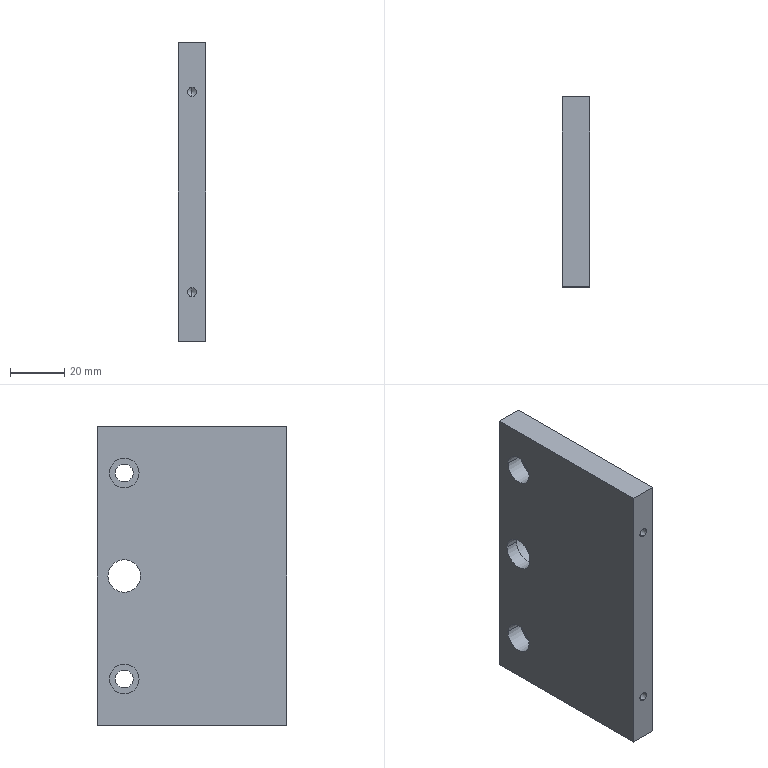Component | SolidWorks | CS021-A10-A003-1 | 1 solid | 29 faces | box 10 x 70 x 110 mm | volume 73715 mm3 | cylinder 16 | plane 9 | cone 4 | commonest cylinder face diameters 11 x4 6.6 x4 3.3 x4 12 x2 16 x2 | material AL6061
build123d program:
from build123d import *

# Parameters (mm, degrees)
SKETCH1_W                                          = 110
SKETCH1_H                                          = 70
BOSS_EXTRUDE1_DEPTH                                = 5
M4_TAPPED_HOLE1_D                                  = 3.3
M4_TAPPED_HOLE1_DEPTH                              = 11.5
M4_TAPPED_HOLE1_TIP                                = 0.9914
HOLE_SIZE_ACCORDING_TO_SLOTTED_PAN_HEA_D           = 6.6
HOLE_SIZE_ACCORDING_TO_SLOTTED_PAN_HEA_CBORE_D     = 11
HOLE_SIZE_ACCORDING_TO_SLOTTED_PAN_HEA_CBORE_DEPTH = 6.8
SKETCH6_R                                          = 8
CUT_EXTRUDE1_DEPTH                                 = 5
SKETCH7_R                                          = 6
CUT_EXTRUDE2_DEPTH                                 = 66.383


with BuildPart() as part:
    # Sketch1 → Boss-Extrude1 (new, symmetric)
    with BuildSketch(Plane(origin=(0, 0, 0), x_dir=(1, 0, 0), z_dir=(0, 1, 0))):
        Rectangle(SKETCH1_W, SKETCH1_H)
    extrude(amount=BOSS_EXTRUDE1_DEPTH, both=True)

    # M4 Tapped Hole1
    with Locations(Plane.XY.offset(35)):
        with Locations((-37, 0), (37, 0)):
            Hole(M4_TAPPED_HOLE1_D / 2, depth=M4_TAPPED_HOLE1_DEPTH)
            with Locations((0, 0, -(M4_TAPPED_HOLE1_DEPTH + M4_TAPPED_HOLE1_TIP / 2))):  # 118° drill point
                Cone(0, M4_TAPPED_HOLE1_D / 2, M4_TAPPED_HOLE1_TIP, mode=Mode.SUBTRACT)

    # Hole Size _according to_ Slotted Pan Hea (through all)
    with Locations(Plane(origin=(0, 5, 0), x_dir=(1, 0, 0), z_dir=(0, 1, 0))):
        with Locations((-38, 25), (38, 25)):
            CounterBoreHole(HOLE_SIZE_ACCORDING_TO_SLOTTED_PAN_HEA_D / 2, HOLE_SIZE_ACCORDING_TO_SLOTTED_PAN_HEA_CBORE_D / 2, HOLE_SIZE_ACCORDING_TO_SLOTTED_PAN_HEA_CBORE_DEPTH)

    # Sketch6 → Cut-Extrude1 (cut)
    with BuildSketch(Plane.XZ.offset(5)):
        with Locations(Location((0, -25, 0), (0, 0, 270))):
            Circle(SKETCH6_R)
    extrude(amount=-CUT_EXTRUDE1_DEPTH, mode=Mode.SUBTRACT)

    # Sketch7 → Cut-Extrude2 (cut, through all)
    with BuildSketch(Plane.XZ):
        with Locations(Location((0, -25, 0), (0, 0, 270))):
            Circle(SKETCH7_R)
    extrude(amount=-CUT_EXTRUDE2_DEPTH, mode=Mode.SUBTRACT)


solid = part.part

# Placed as in the assembly
solid = solid.moved(Location((-159.051, 59.817, 0), (90, 0, 90)))
STEP:
#1=COLOUR_RGB('',0.7922,0.8196,0.9333);
#2=FILL_AREA_STYLE_COLOUR('',#1);
#3=FILL_AREA_STYLE('',(#2));
#4=SURFACE_STYLE_FILL_AREA(#3);
#5=SURFACE_SIDE_STYLE('',(#4));
#6=SURFACE_STYLE_USAGE(.BOTH.,#5);
#7=PRESENTATION_STYLE_ASSIGNMENT((#6));
#8=CARTESIAN_POINT('',(-6.459,3.103,-0.));
#9=VERTEX_POINT('',#8);
#10=CARTESIAN_POINT('',(-6.459,3.575,-0.));
#11=VERTEX_POINT('',#10);
#12=CARTESIAN_POINT('',(-6.459,3.339,-0.));
#13=DIRECTION('',(1.,-0.,0.));
#14=DIRECTION('',(0.,1.,0.));
#15=AXIS2_PLACEMENT_3D('',#12,#13,#14);
#16=CIRCLE('',#15,0.2362);
#17=EDGE_CURVE('',#9,#11,#16,.T.);
#18=ORIENTED_EDGE('',*,*,#17,.F.);
#19=CARTESIAN_POINT('',(-6.262,3.103,-0.));
#20=VERTEX_POINT('',#19);
#21=CARTESIAN_POINT('',(-6.459,3.103,-0.));
#22=DIRECTION('',(1.,-0.,0.));
#23=VECTOR('',#22,39.37);
#24=LINE('',#21,#23);
#25=EDGE_CURVE('',#9,#20,#24,.T.);
#26=ORIENTED_EDGE('',*,*,#25,.T.);
#27=CARTESIAN_POINT('',(-6.262,3.575,-0.));
#28=VERTEX_POINT('',#27);
#29=CARTESIAN_POINT('',(-6.262,3.339,-0.));
#30=DIRECTION('',(1.,-0.,0.));
#31=DIRECTION('',(0.,1.,0.));
#32=AXIS2_PLACEMENT_3D('',#29,#30,#31);
#33=CIRCLE('',#32,0.2362);
#34=EDGE_CURVE('',#20,#28,#33,.T.);
#35=ORIENTED_EDGE('',*,*,#34,.T.);
#36=CARTESIAN_POINT('',(-6.459,3.575,-0.));
#37=DIRECTION('',(1.,-0.,0.));
#38=VECTOR('',#37,39.37);
#39=LINE('',#36,#38);
#40=EDGE_CURVE('',#11,#28,#39,.T.);
#41=ORIENTED_EDGE('',*,*,#40,.F.);
#42=EDGE_LOOP('',(#18,#26,#35,#41));
#43=FACE_OUTER_BOUND('',#42,.T.);
#44=CARTESIAN_POINT('',(-6.459,3.339,-0.));
#45=DIRECTION('',(1.,-0.,0.));
#46=DIRECTION('',(0.,1.,0.));
#47=AXIS2_PLACEMENT_3D('',#44,#45,#46);
#48=CYLINDRICAL_SURFACE('',#47,0.2362);
#49=ADVANCED_FACE('',(#43),#48,.F.);
#50=CARTESIAN_POINT('',(-6.262,3.024,-0.));
#51=VERTEX_POINT('',#50);
#52=CARTESIAN_POINT('',(-6.262,3.654,-0.));
#53=VERTEX_POINT('',#52);
#54=CARTESIAN_POINT('',(-6.262,3.339,-0.));
#55=DIRECTION('',(1.,-0.,0.));
#56=DIRECTION('',(0.,1.,0.));
#57=AXIS2_PLACEMENT_3D('',#54,#55,#56);
#58=CIRCLE('',#57,0.315);
#59=EDGE_CURVE('',#51,#53,#58,.T.);
#60=ORIENTED_EDGE('',*,*,#59,.F.);
#61=CARTESIAN_POINT('',(-6.065,3.024,-0.));
#62=VERTEX_POINT('',#61);
#63=CARTESIAN_POINT('',(-6.262,3.024,-0.));
#64=DIRECTION('',(1.,-0.,0.));
#65=VECTOR('',#64,39.37);
#66=LINE('',#63,#65);
#67=EDGE_CURVE('',#51,#62,#66,.T.);
#68=ORIENTED_EDGE('',*,*,#67,.T.);
#69=CARTESIAN_POINT('',(-6.065,3.654,-0.));
#70=VERTEX_POINT('',#69);
#71=CARTESIAN_POINT('',(-6.065,3.339,-0.));
#72=DIRECTION('',(1.,-0.,0.));
#73=DIRECTION('',(0.,1.,0.));
#74=AXIS2_PLACEMENT_3D('',#71,#72,#73);
#75=CIRCLE('',#74,0.315);
#76=EDGE_CURVE('',#62,#70,#75,.T.);
#77=ORIENTED_EDGE('',*,*,#76,.T.);
#78=CARTESIAN_POINT('',(-6.262,3.654,-0.));
#79=DIRECTION('',(1.,-0.,0.));
#80=VECTOR('',#79,39.37);
#81=LINE('',#78,#80);
#82=EDGE_CURVE('',#53,#70,#81,.T.);
#83=ORIENTED_EDGE('',*,*,#82,.F.);
#84=EDGE_LOOP('',(#60,#68,#77,#83));
#85=FACE_OUTER_BOUND('',#84,.T.);
#86=CARTESIAN_POINT('',(-6.262,3.339,-0.));
#87=DIRECTION('',(1.,-0.,0.));
#88=DIRECTION('',(0.,1.,0.));
#89=AXIS2_PLACEMENT_3D('',#86,#87,#88);
#90=CYLINDRICAL_SURFACE('',#89,0.315);
#91=ADVANCED_FACE('',(#85),#90,.F.);
#92=CARTESIAN_POINT('',(-6.191,3.556,-1.496));
#93=VERTEX_POINT('',#92);
#94=CARTESIAN_POINT('',(-6.191,3.123,-1.496));
#95=VERTEX_POINT('',#94);
#96=CARTESIAN_POINT('',(-6.191,3.339,-1.496));
#97=DIRECTION('',(-1.,0.,0.));
#98=DIRECTION('',(0.,-1.,0.));
#99=AXIS2_PLACEMENT_3D('',#96,#97,#98);
#100=CIRCLE('',#99,0.2165);
#101=EDGE_CURVE('',#93,#95,#100,.T.);
#102=ORIENTED_EDGE('',*,*,#101,.F.);
#103=CARTESIAN_POINT('',(-6.459,3.556,-1.496));
#104=VERTEX_POINT('',#103);
#105=CARTESIAN_POINT('',(-6.459,3.556,-1.496));
#106=DIRECTION('',(-1.,0.,0.));
#107=VECTOR('',#106,39.37);
#108=LINE('',#105,#107);
#109=EDGE_CURVE('',#93,#104,#108,.T.);
#110=ORIENTED_EDGE('',*,*,#109,.T.);
#111=CARTESIAN_POINT('',(-6.459,3.123,-1.496));
#112=VERTEX_POINT('',#111);
#113=CARTESIAN_POINT('',(-6.459,3.339,-1.496));
#114=DIRECTION('',(-1.,0.,0.));
#115=DIRECTION('',(0.,-1.,0.));
#116=AXIS2_PLACEMENT_3D('',#113,#114,#115);
#117=CIRCLE('',#116,0.2165);
#118=EDGE_CURVE('',#104,#112,#117,.T.);
#119=ORIENTED_EDGE('',*,*,#118,.T.);
#120=CARTESIAN_POINT('',(-6.459,3.123,-1.496));
#121=DIRECTION('',(-1.,0.,0.));
#122=VECTOR('',#121,39.37);
#123=LINE('',#120,#122);
#124=EDGE_CURVE('',#95,#112,#123,.T.);
#125=ORIENTED_EDGE('',*,*,#124,.F.);
#126=EDGE_LOOP('',(#102,#110,#119,#125));
#127=FACE_OUTER_BOUND('',#126,.T.);
#128=CARTESIAN_POINT('',(-6.459,3.339,-1.496));
#129=DIRECTION('',(-1.,0.,0.));
#130=DIRECTION('',(0.,-1.,0.));
#131=AXIS2_PLACEMENT_3D('',#128,#129,#130);
#132=CYLINDRICAL_SURFACE('',#131,0.2165);
#133=ADVANCED_FACE('',(#127),#132,.F.);
#134=CARTESIAN_POINT('',(-6.065,3.469,-1.496));
#135=VERTEX_POINT('',#134);
#136=CARTESIAN_POINT('',(-6.065,3.209,-1.496));
#137=VERTEX_POINT('',#136);
#138=CARTESIAN_POINT('',(-6.065,3.339,-1.496));
#139=DIRECTION('',(-1.,0.,0.));
#140=DIRECTION('',(0.,-1.,0.));
#141=AXIS2_PLACEMENT_3D('',#138,#139,#140);
#142=CIRCLE('',#141,0.1299);
#143=EDGE_CURVE('',#135,#137,#142,.T.);
#144=ORIENTED_EDGE('',*,*,#143,.F.);
#145=CARTESIAN_POINT('',(-6.191,3.469,-1.496));
#146=VERTEX_POINT('',#145);
#147=CARTESIAN_POINT('',(-6.459,3.469,-1.496));
#148=DIRECTION('',(-1.,0.,0.));
#149=VECTOR('',#148,39.37);
#150=LINE('',#147,#149);
#151=EDGE_CURVE('',#135,#146,#150,.T.);
#152=ORIENTED_EDGE('',*,*,#151,.T.);
#153=CARTESIAN_POINT('',(-6.191,3.209,-1.496));
#154=VERTEX_POINT('',#153);
#155=CARTESIAN_POINT('',(-6.191,3.339,-1.496));
#156=DIRECTION('',(-1.,0.,0.));
#157=DIRECTION('',(0.,-1.,0.));
#158=AXIS2_PLACEMENT_3D('',#155,#156,#157);
#159=CIRCLE('',#158,0.1299);
#160=EDGE_CURVE('',#146,#154,#159,.T.);
#161=ORIENTED_EDGE('',*,*,#160,.T.);
#162=CARTESIAN_POINT('',(-6.459,3.209,-1.496));
#163=DIRECTION('',(-1.,0.,0.));
#164=VECTOR('',#163,39.37);
#165=LINE('',#162,#164);
#166=EDGE_CURVE('',#137,#154,#165,.T.);
#167=ORIENTED_EDGE('',*,*,#166,.F.);
#168=EDGE_LOOP('',(#144,#152,#161,#167));
#169=FACE_OUTER_BOUND('',#168,.T.);
#170=CARTESIAN_POINT('',(-6.459,3.339,-1.496));
#171=DIRECTION('',(-1.,0.,0.));
#172=DIRECTION('',(0.,-1.,0.));
#173=AXIS2_PLACEMENT_3D('',#170,#171,#172);
#174=CYLINDRICAL_SURFACE('',#173,0.1299);
#175=ADVANCED_FACE('',(#169),#174,.F.);
#176=CARTESIAN_POINT('',(-6.191,3.556,1.496));
#177=VERTEX_POINT('',#176);
#178=CARTESIAN_POINT('',(-6.191,3.123,1.496));
#179=VERTEX_POINT('',#178);
#180=CARTESIAN_POINT('',(-6.191,3.339,1.496));
#181=DIRECTION('',(-1.,0.,0.));
#182=DIRECTION('',(0.,-1.,0.));
#183=AXIS2_PLACEMENT_3D('',#180,#181,#182);
#184=CIRCLE('',#183,0.2165);
#185=EDGE_CURVE('',#177,#179,#184,.T.);
#186=ORIENTED_EDGE('',*,*,#185,.F.);
#187=CARTESIAN_POINT('',(-6.459,3.556,1.496));
#188=VERTEX_POINT('',#187);
#189=CARTESIAN_POINT('',(-6.459,3.556,1.496));
#190=DIRECTION('',(-1.,0.,0.));
#191=VECTOR('',#190,39.37);
#192=LINE('',#189,#191);
#193=EDGE_CURVE('',#177,#188,#192,.T.);
#194=ORIENTED_EDGE('',*,*,#193,.T.);
#195=CARTESIAN_POINT('',(-6.459,3.123,1.496));
#196=VERTEX_POINT('',#195);
#197=CARTESIAN_POINT('',(-6.459,3.339,1.496));
#198=DIRECTION('',(-1.,0.,0.));
#199=DIRECTION('',(0.,-1.,0.));
#200=AXIS2_PLACEMENT_3D('',#197,#198,#199);
#201=CIRCLE('',#200,0.2165);
#202=EDGE_CURVE('',#188,#196,#201,.T.);
#203=ORIENTED_EDGE('',*,*,#202,.T.);
#204=CARTESIAN_POINT('',(-6.459,3.123,1.496));
#205=DIRECTION('',(-1.,0.,0.));
#206=VECTOR('',#205,39.37);
#207=LINE('',#204,#206);
#208=EDGE_CURVE('',#179,#196,#207,.T.);
#209=ORIENTED_EDGE('',*,*,#208,.F.);
#210=EDGE_LOOP('',(#186,#194,#203,#209));
#211=FACE_OUTER_BOUND('',#210,.T.);
#212=CARTESIAN_POINT('',(-6.459,3.339,1.496));
#213=DIRECTION('',(-1.,0.,0.));
#214=DIRECTION('',(0.,-1.,0.));
#215=AXIS2_PLACEMENT_3D('',#212,#213,#214);
#216=CYLINDRICAL_SURFACE('',#215,0.2165);
#217=ADVANCED_FACE('',(#211),#216,.F.);
#218=CARTESIAN_POINT('',(-6.065,3.469,1.496));
#219=VERTEX_POINT('',#218);
#220=CARTESIAN_POINT('',(-6.065,3.209,1.496));
#221=VERTEX_POINT('',#220);
#222=CARTESIAN_POINT('',(-6.065,3.339,1.496));
#223=DIRECTION('',(-1.,0.,0.));
#224=DIRECTION('',(0.,-1.,0.));
#225=AXIS2_PLACEMENT_3D('',#222,#223,#224);
#226=CIRCLE('',#225,0.1299);
#227=EDGE_CURVE('',#219,#221,#226,.T.);
#228=ORIENTED_EDGE('',*,*,#227,.F.);
#229=CARTESIAN_POINT('',(-6.191,3.469,1.496));
#230=VERTEX_POINT('',#229);
#231=CARTESIAN_POINT('',(-6.459,3.469,1.496));
#232=DIRECTION('',(-1.,0.,0.));
#233=VECTOR('',#232,39.37);
#234=LINE('',#231,#233);
#235=EDGE_CURVE('',#219,#230,#234,.T.);
#236=ORIENTED_EDGE('',*,*,#235,.T.);
#237=CARTESIAN_POINT('',(-6.191,3.209,1.496));
#238=VERTEX_POINT('',#237);
#239=CARTESIAN_POINT('',(-6.191,3.339,1.496));
#240=DIRECTION('',(-1.,0.,0.));
#241=DIRECTION('',(0.,-1.,0.));
#242=AXIS2_PLACEMENT_3D('',#239,#240,#241);
#243=CIRCLE('',#242,0.1299);
#244=EDGE_CURVE('',#230,#238,#243,.T.);
#245=ORIENTED_EDGE('',*,*,#244,.T.);
#246=CARTESIAN_POINT('',(-6.459,3.209,1.496));
#247=DIRECTION('',(-1.,0.,0.));
#248=VECTOR('',#247,39.37);
#249=LINE('',#246,#248);
#250=EDGE_CURVE('',#221,#238,#249,.T.);
#251=ORIENTED_EDGE('',*,*,#250,.F.);
#252=EDGE_LOOP('',(#228,#236,#245,#251));
#253=FACE_OUTER_BOUND('',#252,.T.);
#254=CARTESIAN_POINT('',(-6.459,3.339,1.496));
#255=DIRECTION('',(-1.,0.,0.));
#256=DIRECTION('',(0.,-1.,0.));
#257=AXIS2_PLACEMENT_3D('',#254,#255,#256);
#258=CYLINDRICAL_SURFACE('',#257,0.1299);
#259=ADVANCED_FACE('',(#253),#258,.F.);
#260=CARTESIAN_POINT('',(-6.262,1.43,-1.522));
#261=VERTEX_POINT('',#260);
#262=CARTESIAN_POINT('',(-6.262,1.43,-1.392));
#263=VERTEX_POINT('',#262);
#264=CARTESIAN_POINT('',(-6.262,1.43,-1.457));
#265=DIRECTION('',(-0.,-1.,-0.));
#266=DIRECTION('',(0.,0.,1.));
#267=AXIS2_PLACEMENT_3D('',#264,#265,#266);
#268=CIRCLE('',#267,0.06496);
#269=EDGE_CURVE('',#261,#263,#268,.T.);
#270=ORIENTED_EDGE('',*,*,#269,.F.);
#271=CARTESIAN_POINT('',(-6.262,0.977,-1.522));
#272=VERTEX_POINT('',#271);
#273=CARTESIAN_POINT('',(-6.262,0.977,-1.522));
#274=DIRECTION('',(-0.,-1.,-0.));
#275=VECTOR('',#274,39.37);
#276=LINE('',#273,#275);
#277=EDGE_CURVE('',#261,#272,#276,.T.);
#278=ORIENTED_EDGE('',*,*,#277,.T.);
#279=CARTESIAN_POINT('',(-6.262,0.977,-1.392));
#280=VERTEX_POINT('',#279);
#281=CARTESIAN_POINT('',(-6.262,0.977,-1.457));
#282=DIRECTION('',(-0.,-1.,-0.));
#283=DIRECTION('',(0.,0.,1.));
#284=AXIS2_PLACEMENT_3D('',#281,#282,#283);
#285=CIRCLE('',#284,0.06496);
#286=EDGE_CURVE('',#272,#280,#285,.T.);
#287=ORIENTED_EDGE('',*,*,#286,.T.);
#288=CARTESIAN_POINT('',(-6.262,0.977,-1.392));
#289=DIRECTION('',(-0.,-1.,-0.));
#290=VECTOR('',#289,39.37);
#291=LINE('',#288,#290);
#292=EDGE_CURVE('',#263,#280,#291,.T.);
#293=ORIENTED_EDGE('',*,*,#292,.F.);
#294=EDGE_LOOP('',(#270,#278,#287,#293));
#295=FACE_OUTER_BOUND('',#294,.T.);
#296=CARTESIAN_POINT('',(-6.262,0.977,-1.457));
#297=DIRECTION('',(-0.,-1.,-0.));
#298=DIRECTION('',(0.,0.,1.));
#299=AXIS2_PLACEMENT_3D('',#296,#297,#298);
#300=CYLINDRICAL_SURFACE('',#299,0.06496);
#301=ADVANCED_FACE('',(#295),#300,.F.);
#302=CARTESIAN_POINT('',(-6.262,1.469,-1.457));
#303=VERTEX_POINT('',#302);
#304=CARTESIAN_POINT('',(-6.262,1.43,-1.392));
#305=DIRECTION('',(-0.,-0.515,0.8572));
#306=VECTOR('',#305,39.37);
#307=LINE('',#304,#306);
#308=EDGE_CURVE('',#303,#263,#307,.T.);
#309=ORIENTED_EDGE('',*,*,#308,.F.);
#310=CARTESIAN_POINT('',(-6.262,1.43,-1.522));
#311=DIRECTION('',(-0.,-0.515,-0.8572));
#312=VECTOR('',#311,39.37);
#313=LINE('',#310,#312);
#314=EDGE_CURVE('',#303,#261,#313,.T.);
#315=ORIENTED_EDGE('',*,*,#314,.T.);
#316=ORIENTED_EDGE('',*,*,#269,.T.);
#317=EDGE_LOOP('',(#309,#315,#316));
#318=FACE_OUTER_BOUND('',#317,.T.);
#319=CARTESIAN_POINT('',(-6.262,1.43,-1.457));
#320=DIRECTION('',(-0.,-1.,-0.));
#321=DIRECTION('',(0.,0.,1.));
#322=AXIS2_PLACEMENT_3D('',#319,#320,#321);
#323=CONICAL_SURFACE('',#322,0.06496,1.03);
#324=ADVANCED_FACE('',(#318),#323,.F.);
#325=CARTESIAN_POINT('',(-6.262,1.43,1.392));
#326=VERTEX_POINT('',#325);
#327=CARTESIAN_POINT('',(-6.262,1.43,1.522));
#328=VERTEX_POINT('',#327);
#329=CARTESIAN_POINT('',(-6.262,1.43,1.457));
#330=DIRECTION('',(-0.,-1.,-0.));
#331=DIRECTION('',(0.,0.,1.));
#332=AXIS2_PLACEMENT_3D('',#329,#330,#331);
#333=CIRCLE('',#332,0.06496);
#334=EDGE_CURVE('',#326,#328,#333,.T.);
#335=ORIENTED_EDGE('',*,*,#334,.F.);
#336=CARTESIAN_POINT('',(-6.262,0.977,1.392));
#337=VERTEX_POINT('',#336);
#338=CARTESIAN_POINT('',(-6.262,0.977,1.392));
#339=DIRECTION('',(-0.,-1.,-0.));
#340=VECTOR('',#339,39.37);
#341=LINE('',#338,#340);
#342=EDGE_CURVE('',#326,#337,#341,.T.);
#343=ORIENTED_EDGE('',*,*,#342,.T.);
#344=CARTESIAN_POINT('',(-6.262,0.977,1.522));
#345=VERTEX_POINT('',#344);
#346=CARTESIAN_POINT('',(-6.262,0.977,1.457));
#347=DIRECTION('',(-0.,-1.,-0.));
#348=DIRECTION('',(0.,0.,1.));
#349=AXIS2_PLACEMENT_3D('',#346,#347,#348);
#350=CIRCLE('',#349,0.06496);
#351=EDGE_CURVE('',#337,#345,#350,.T.);
#352=ORIENTED_EDGE('',*,*,#351,.T.);
#353=CARTESIAN_POINT('',(-6.262,0.977,1.522));
#354=DIRECTION('',(-0.,-1.,-0.));
#355=VECTOR('',#354,39.37);
#356=LINE('',#353,#355);
#357=EDGE_CURVE('',#328,#345,#356,.T.);
#358=ORIENTED_EDGE('',*,*,#357,.F.);
#359=EDGE_LOOP('',(#335,#343,#352,#358));
#360=FACE_OUTER_BOUND('',#359,.T.);
#361=CARTESIAN_POINT('',(-6.262,0.977,1.457));
#362=DIRECTION('',(-0.,-1.,-0.));
#363=DIRECTION('',(0.,0.,1.));
#364=AXIS2_PLACEMENT_3D('',#361,#362,#363);
#365=CYLINDRICAL_SURFACE('',#364,0.06496);
#366=ADVANCED_FACE('',(#360),#365,.F.);
#367=CARTESIAN_POINT('',(-6.262,1.469,1.457));
#368=VERTEX_POINT('',#367);
#369=CARTESIAN_POINT('',(-6.262,1.43,1.522));
#370=DIRECTION('',(-0.,-0.515,0.8572));
#371=VECTOR('',#370,39.37);
#372=LINE('',#369,#371);
#373=EDGE_CURVE('',#368,#328,#372,.T.);
#374=ORIENTED_EDGE('',*,*,#373,.F.);
#375=CARTESIAN_POINT('',(-6.262,1.43,1.392));
#376=DIRECTION('',(-0.,-0.515,-0.8572));
#377=VECTOR('',#376,39.37);
#378=LINE('',#375,#377);
#379=EDGE_CURVE('',#368,#326,#378,.T.);
#380=ORIENTED_EDGE('',*,*,#379,.T.);
#381=ORIENTED_EDGE('',*,*,#334,.T.);
#382=EDGE_LOOP('',(#374,#380,#381));
#383=FACE_OUTER_BOUND('',#382,.T.);
#384=CARTESIAN_POINT('',(-6.262,1.43,1.457));
#385=DIRECTION('',(-0.,-1.,-0.));
#386=DIRECTION('',(0.,0.,1.));
#387=AXIS2_PLACEMENT_3D('',#384,#385,#386);
#388=CONICAL_SURFACE('',#387,0.06496,1.03);
#389=ADVANCED_FACE('',(#383),#388,.F.);
#390=CARTESIAN_POINT('',(-6.065,0.977,2.165));
#391=VERTEX_POINT('',#390);
#392=CARTESIAN_POINT('',(-6.065,3.733,2.165));
#393=VERTEX_POINT('',#392);
#394=CARTESIAN_POINT('',(-6.065,0.977,2.165));
#395=DIRECTION('',(0.,1.,0.));
#396=VECTOR('',#395,39.37);
#397=LINE('',#394,#396);
#398=EDGE_CURVE('',#391,#393,#397,.T.);
#399=ORIENTED_EDGE('',*,*,#398,.T.);
#400=CARTESIAN_POINT('',(-6.459,3.733,2.165));
#401=VERTEX_POINT('',#400);
#402=CARTESIAN_POINT('',(-6.459,3.733,2.165));
#403=DIRECTION('',(1.,-0.,0.));
#404=VECTOR('',#403,39.37);
#405=LINE('',#402,#404);
#406=EDGE_CURVE('',#401,#393,#405,.T.);
#407=ORIENTED_EDGE('',*,*,#406,.F.);
#408=CARTESIAN_POINT('',(-6.459,0.977,2.165));
#409=VERTEX_POINT('',#408);
#410=CARTESIAN_POINT('',(-6.459,0.977,2.165));
#411=DIRECTION('',(0.,1.,0.));
#412=VECTOR('',#411,39.37);
#413=LINE('',#410,#412);
#414=EDGE_CURVE('',#409,#401,#413,.T.);
#415=ORIENTED_EDGE('',*,*,#414,.F.);
#416=CARTESIAN_POINT('',(-6.459,0.977,2.165));
#417=DIRECTION('',(1.,-0.,0.));
#418=VECTOR('',#417,39.37);
#419=LINE('',#416,#418);
#420=EDGE_CURVE('',#409,#391,#419,.T.);
#421=ORIENTED_EDGE('',*,*,#420,.T.);
#422=EDGE_LOOP('',(#399,#407,#415,#421));
#423=FACE_OUTER_BOUND('',#422,.T.);
#424=CARTESIAN_POINT('',(-6.459,0.977,2.165));
#425=DIRECTION('',(0.,0.,-1.));
#426=DIRECTION('',(-0.,-1.,-0.));
#427=AXIS2_PLACEMENT_3D('',#424,#425,#426);
#428=PLANE('',#427);
#429=ADVANCED_FACE('',(#423),#428,.F.);
#430=CARTESIAN_POINT('',(-6.065,3.733,-2.165));
#431=VERTEX_POINT('',#430);
#432=CARTESIAN_POINT('',(-6.065,3.733,-2.165));
#433=DIRECTION('',(0.,0.,-1.));
#434=VECTOR('',#433,39.37);
#435=LINE('',#432,#434);
#436=EDGE_CURVE('',#393,#431,#435,.T.);
#437=ORIENTED_EDGE('',*,*,#436,.T.);
#438=CARTESIAN_POINT('',(-6.459,3.733,-2.165));
#439=VERTEX_POINT('',#438);
#440=CARTESIAN_POINT('',(-6.459,3.733,-2.165));
#441=DIRECTION('',(1.,-0.,0.));
#442=VECTOR('',#441,39.37);
#443=LINE('',#440,#442);
#444=EDGE_CURVE('',#439,#431,#443,.T.);
#445=ORIENTED_EDGE('',*,*,#444,.F.);
#446=CARTESIAN_POINT('',(-6.459,3.733,-2.165));
#447=DIRECTION('',(0.,0.,-1.));
#448=VECTOR('',#447,39.37);
#449=LINE('',#446,#448);
#450=EDGE_CURVE('',#401,#439,#449,.T.);
#451=ORIENTED_EDGE('',*,*,#450,.F.);
#452=ORIENTED_EDGE('',*,*,#406,.T.);
#453=EDGE_LOOP('',(#437,#445,#451,#452));
#454=FACE_OUTER_BOUND('',#453,.T.);
#455=CARTESIAN_POINT('',(-6.459,3.733,-2.165));
#456=DIRECTION('',(-0.,-1.,-0.));
#457=DIRECTION('',(-0.,-0.,1.));
#458=AXIS2_PLACEMENT_3D('',#455,#456,#457);
#459=PLANE('',#458);
#460=ADVANCED_FACE('',(#454),#459,.F.);
#461=CARTESIAN_POINT('',(-6.065,0.977,-2.165));
#462=VERTEX_POINT('',#461);
#463=CARTESIAN_POINT('',(-6.065,0.977,-2.165));
#464=DIRECTION('',(-0.,-1.,-0.));
#465=VECTOR('',#464,39.37);
#466=LINE('',#463,#465);
#467=EDGE_CURVE('',#431,#462,#466,.T.);
#468=ORIENTED_EDGE('',*,*,#467,.T.);
#469=CARTESIAN_POINT('',(-6.459,0.977,-2.165));
#470=VERTEX_POINT('',#469);
#471=CARTESIAN_POINT('',(-6.459,0.977,-2.165));
#472=DIRECTION('',(1.,-0.,0.));
#473=VECTOR('',#472,39.37);
#474=LINE('',#471,#473);
#475=EDGE_CURVE('',#470,#462,#474,.T.);
#476=ORIENTED_EDGE('',*,*,#475,.F.);
#477=CARTESIAN_POINT('',(-6.459,0.977,-2.165));
#478=DIRECTION('',(-0.,-1.,-0.));
#479=VECTOR('',#478,39.37);
#480=LINE('',#477,#479);
#481=EDGE_CURVE('',#439,#470,#480,.T.);
#482=ORIENTED_EDGE('',*,*,#481,.F.);
#483=ORIENTED_EDGE('',*,*,#444,.T.);
#484=EDGE_LOOP('',(#468,#476,#482,#483));
#485=FACE_OUTER_BOUND('',#484,.T.);
#486=CARTESIAN_POINT('',(-6.459,0.977,-2.165));
#487=DIRECTION('',(-0.,-0.,1.));
#488=DIRECTION('',(0.,1.,0.));
#489=AXIS2_PLACEMENT_3D('',#486,#487,#488);
#490=PLANE('',#489);
#491=ADVANCED_FACE('',(#485),#490,.F.);
#492=CARTESIAN_POINT('',(-6.262,0.977,-1.457));
#493=DIRECTION('',(-0.,-1.,-0.));
#494=DIRECTION('',(0.,0.,1.));
#495=AXIS2_PLACEMENT_3D('',#492,#493,#494);
#496=CIRCLE('',#495,0.06496);
#497=EDGE_CURVE('',#280,#272,#496,.T.);
#498=ORIENTED_EDGE('',*,*,#497,.F.);
#499=ORIENTED_EDGE('',*,*,#286,.F.);
#500=EDGE_LOOP('',(#498,#499));
#501=FACE_BOUND('',#500,.T.);
#502=CARTESIAN_POINT('',(-6.262,0.977,1.457));
#503=DIRECTION('',(-0.,-1.,-0.));
#504=DIRECTION('',(0.,0.,1.));
#505=AXIS2_PLACEMENT_3D('',#502,#503,#504);
#506=CIRCLE('',#505,0.06496);
#507=EDGE_CURVE('',#345,#337,#506,.T.);
#508=ORIENTED_EDGE('',*,*,#507,.F.);
#509=ORIENTED_EDGE('',*,*,#351,.F.);
#510=EDGE_LOOP('',(#508,#509));
#511=FACE_BOUND('',#510,.T.);
#512=CARTESIAN_POINT('',(-6.065,0.977,-2.165));
#513=DIRECTION('',(-0.,-0.,1.));
#514=VECTOR('',#513,39.37);
#515=LINE('',#512,#514);
#516=EDGE_CURVE('',#462,#391,#515,.T.);
#517=ORIENTED_EDGE('',*,*,#516,.T.);
#518=ORIENTED_EDGE('',*,*,#420,.F.);
#519=CARTESIAN_POINT('',(-6.459,0.977,-2.165));
#520=DIRECTION('',(-0.,-0.,1.));
#521=VECTOR('',#520,39.37);
#522=LINE('',#519,#521);
#523=EDGE_CURVE('',#470,#409,#522,.T.);
#524=ORIENTED_EDGE('',*,*,#523,.F.);
#525=ORIENTED_EDGE('',*,*,#475,.T.);
#526=EDGE_LOOP('',(#517,#518,#524,#525));
#527=FACE_OUTER_BOUND('',#526,.T.);
#528=CARTESIAN_POINT('',(-6.459,0.977,-2.165));
#529=DIRECTION('',(0.,1.,0.));
#530=DIRECTION('',(0.,0.,-1.));
#531=AXIS2_PLACEMENT_3D('',#528,#529,#530);
#532=PLANE('',#531);
#533=ADVANCED_FACE('',(#501,#511,#527),#532,.F.);
#534=CARTESIAN_POINT('',(-6.459,3.339,-0.));
#535=DIRECTION('',(1.,-0.,0.));
#536=DIRECTION('',(0.,1.,0.));
#537=AXIS2_PLACEMENT_3D('',#534,#535,#536);
#538=CIRCLE('',#537,0.2362);
#539=EDGE_CURVE('',#11,#9,#538,.T.);
#540=ORIENTED_EDGE('',*,*,#539,.T.);
#541=ORIENTED_EDGE('',*,*,#17,.T.);
#542=EDGE_LOOP('',(#540,#541));
#543=FACE_BOUND('',#542,.T.);
#544=CARTESIAN_POINT('',(-6.459,3.339,-1.496));
#545=DIRECTION('',(-1.,0.,0.));
#546=DIRECTION('',(0.,-1.,0.));
#547=AXIS2_PLACEMENT_3D('',#544,#545,#546);
#548=CIRCLE('',#547,0.2165);
#549=EDGE_CURVE('',#112,#104,#548,.T.);
#550=ORIENTED_EDGE('',*,*,#549,.F.);
#551=ORIENTED_EDGE('',*,*,#118,.F.);
#552=EDGE_LOOP('',(#550,#551));
#553=FACE_BOUND('',#552,.T.);
#554=CARTESIAN_POINT('',(-6.459,3.339,1.496));
#555=DIRECTION('',(-1.,0.,0.));
#556=DIRECTION('',(0.,-1.,0.));
#557=AXIS2_PLACEMENT_3D('',#554,#555,#556);
#558=CIRCLE('',#557,0.2165);
#559=EDGE_CURVE('',#196,#188,#558,.T.);
#560=ORIENTED_EDGE('',*,*,#559,.F.);
#561=ORIENTED_EDGE('',*,*,#202,.F.);
#562=EDGE_LOOP('',(#560,#561));
#563=FACE_BOUND('',#562,.T.);
#564=ORIENTED_EDGE('',*,*,#414,.T.);
#565=ORIENTED_EDGE('',*,*,#450,.T.);
#566=ORIENTED_EDGE('',*,*,#481,.T.);
#567=ORIENTED_EDGE('',*,*,#523,.T.);
#568=EDGE_LOOP('',(#564,#565,#566,#567));
#569=FACE_OUTER_BOUND('',#568,.T.);
#570=CARTESIAN_POINT('',(-6.459,2.355,-0.));
#571=DIRECTION('',(1.,-0.,-0.));
#572=DIRECTION('',(0.,1.,0.));
#573=AXIS2_PLACEMENT_3D('',#570,#571,#572);
#574=PLANE('',#573);
#575=ADVANCED_FACE('',(#543,#553,#563,#569),#574,.F.);
#576=CARTESIAN_POINT('',(-6.065,3.339,-0.));
#577=DIRECTION('',(1.,-0.,0.));
#578=DIRECTION('',(0.,1.,0.));
#579=AXIS2_PLACEMENT_3D('',#576,#577,#578);
#580=CIRCLE('',#579,0.315);
#581=EDGE_CURVE('',#70,#62,#580,.T.);
#582=ORIENTED_EDGE('',*,*,#581,.F.);
#583=ORIENTED_EDGE('',*,*,#76,.F.);
#584=EDGE_LOOP('',(#582,#583));
#585=FACE_BOUND('',#584,.T.);
#586=CARTESIAN_POINT('',(-6.065,3.339,-1.496));
#587=DIRECTION('',(-1.,0.,0.));
#588=DIRECTION('',(0.,-1.,0.));
#589=AXIS2_PLACEMENT_3D('',#586,#587,#588);
#590=CIRCLE('',#589,0.1299);
#591=EDGE_CURVE('',#137,#135,#590,.T.);
#592=ORIENTED_EDGE('',*,*,#591,.T.);
#593=ORIENTED_EDGE('',*,*,#143,.T.);
#594=EDGE_LOOP('',(#592,#593));
#595=FACE_BOUND('',#594,.T.);
#596=CARTESIAN_POINT('',(-6.065,3.339,1.496));
#597=DIRECTION('',(-1.,0.,0.));
#598=DIRECTION('',(0.,-1.,0.));
#599=AXIS2_PLACEMENT_3D('',#596,#597,#598);
#600=CIRCLE('',#599,0.1299);
#601=EDGE_CURVE('',#221,#219,#600,.T.);
#602=ORIENTED_EDGE('',*,*,#601,.T.);
#603=ORIENTED_EDGE('',*,*,#227,.T.);
#604=EDGE_LOOP('',(#602,#603));
#605=FACE_BOUND('',#604,.T.);
#606=ORIENTED_EDGE('',*,*,#398,.F.);
#607=ORIENTED_EDGE('',*,*,#516,.F.);
#608=ORIENTED_EDGE('',*,*,#467,.F.);
#609=ORIENTED_EDGE('',*,*,#436,.F.);
#610=EDGE_LOOP('',(#606,#607,#608,#609));
#611=FACE_OUTER_BOUND('',#610,.T.);
#612=CARTESIAN_POINT('',(-6.065,2.355,-0.));
#613=DIRECTION('',(1.,-0.,-0.));
#614=DIRECTION('',(0.,1.,0.));
#615=AXIS2_PLACEMENT_3D('',#612,#613,#614);
#616=PLANE('',#615);
#617=ADVANCED_FACE('',(#585,#595,#605,#611),#616,.T.);
#618=ORIENTED_EDGE('',*,*,#379,.F.);
#619=ORIENTED_EDGE('',*,*,#373,.T.);
#620=CARTESIAN_POINT('',(-6.262,1.43,1.457));
#621=DIRECTION('',(-0.,-1.,-0.));
#622=DIRECTION('',(0.,0.,1.));
#623=AXIS2_PLACEMENT_3D('',#620,#621,#622);
#624=CIRCLE('',#623,0.06496);
#625=EDGE_CURVE('',#328,#326,#624,.T.);
#626=ORIENTED_EDGE('',*,*,#625,.T.);
#627=EDGE_LOOP('',(#618,#619,#626));
#628=FACE_OUTER_BOUND('',#627,.T.);
#629=CARTESIAN_POINT('',(-6.262,1.43,1.457));
#630=DIRECTION('',(-0.,-1.,-0.));
#631=DIRECTION('',(0.,0.,1.));
#632=AXIS2_PLACEMENT_3D('',#629,#630,#631);
#633=CONICAL_SURFACE('',#632,0.06496,1.03);
#634=ADVANCED_FACE('',(#628),#633,.F.);
#635=ORIENTED_EDGE('',*,*,#342,.F.);
#636=ORIENTED_EDGE('',*,*,#625,.F.);
#637=ORIENTED_EDGE('',*,*,#357,.T.);
#638=ORIENTED_EDGE('',*,*,#507,.T.);
#639=EDGE_LOOP('',(#635,#636,#637,#638));
#640=FACE_OUTER_BOUND('',#639,.T.);
#641=CARTESIAN_POINT('',(-6.262,0.977,1.457));
#642=DIRECTION('',(-0.,-1.,-0.));
#643=DIRECTION('',(0.,0.,1.));
#644=AXIS2_PLACEMENT_3D('',#641,#642,#643);
#645=CYLINDRICAL_SURFACE('',#644,0.06496);
#646=ADVANCED_FACE('',(#640),#645,.F.);
#647=ORIENTED_EDGE('',*,*,#314,.F.);
#648=ORIENTED_EDGE('',*,*,#308,.T.);
#649=CARTESIAN_POINT('',(-6.262,1.43,-1.457));
#650=DIRECTION('',(-0.,-1.,-0.));
#651=DIRECTION('',(0.,0.,1.));
#652=AXIS2_PLACEMENT_3D('',#649,#650,#651);
#653=CIRCLE('',#652,0.06496);
#654=EDGE_CURVE('',#263,#261,#653,.T.);
#655=ORIENTED_EDGE('',*,*,#654,.T.);
#656=EDGE_LOOP('',(#647,#648,#655));
#657=FACE_OUTER_BOUND('',#656,.T.);
#658=CARTESIAN_POINT('',(-6.262,1.43,-1.457));
#659=DIRECTION('',(-0.,-1.,-0.));
#660=DIRECTION('',(0.,0.,1.));
#661=AXIS2_PLACEMENT_3D('',#658,#659,#660);
#662=CONICAL_SURFACE('',#661,0.06496,1.03);
#663=ADVANCED_FACE('',(#657),#662,.F.);
#664=ORIENTED_EDGE('',*,*,#277,.F.);
#665=ORIENTED_EDGE('',*,*,#654,.F.);
#666=ORIENTED_EDGE('',*,*,#292,.T.);
#667=ORIENTED_EDGE('',*,*,#497,.T.);
#668=EDGE_LOOP('',(#664,#665,#666,#667));
#669=FACE_OUTER_BOUND('',#668,.T.);
#670=CARTESIAN_POINT('',(-6.262,0.977,-1.457));
#671=DIRECTION('',(-0.,-1.,-0.));
#672=DIRECTION('',(0.,0.,1.));
#673=AXIS2_PLACEMENT_3D('',#670,#671,#672);
#674=CYLINDRICAL_SURFACE('',#673,0.06496);
#675=ADVANCED_FACE('',(#669),#674,.F.);
#676=ORIENTED_EDGE('',*,*,#235,.F.);
#677=ORIENTED_EDGE('',*,*,#601,.F.);
#678=ORIENTED_EDGE('',*,*,#250,.T.);
#679=CARTESIAN_POINT('',(-6.191,3.339,1.496));
#680=DIRECTION('',(-1.,0.,0.));
#681=DIRECTION('',(0.,-1.,0.));
#682=AXIS2_PLACEMENT_3D('',#679,#680,#681);
#683=CIRCLE('',#682,0.1299);
#684=EDGE_CURVE('',#238,#230,#683,.T.);
#685=ORIENTED_EDGE('',*,*,#684,.T.);
#686=EDGE_LOOP('',(#676,#677,#678,#685));
#687=FACE_OUTER_BOUND('',#686,.T.);
#688=CARTESIAN_POINT('',(-6.459,3.339,1.496));
#689=DIRECTION('',(-1.,0.,0.));
#690=DIRECTION('',(0.,-1.,0.));
#691=AXIS2_PLACEMENT_3D('',#688,#689,#690);
#692=CYLINDRICAL_SURFACE('',#691,0.1299);
#693=ADVANCED_FACE('',(#687),#692,.F.);
#694=ORIENTED_EDGE('',*,*,#684,.F.);
#695=ORIENTED_EDGE('',*,*,#244,.F.);
#696=EDGE_LOOP('',(#694,#695));
#697=FACE_BOUND('',#696,.T.);
#698=CARTESIAN_POINT('',(-6.191,3.339,1.496));
#699=DIRECTION('',(-1.,0.,0.));
#700=DIRECTION('',(0.,-1.,0.));
#701=AXIS2_PLACEMENT_3D('',#698,#699,#700);
#702=CIRCLE('',#701,0.2165);
#703=EDGE_CURVE('',#179,#177,#702,.T.);
#704=ORIENTED_EDGE('',*,*,#703,.T.);
#705=ORIENTED_EDGE('',*,*,#185,.T.);
#706=EDGE_LOOP('',(#704,#705));
#707=FACE_OUTER_BOUND('',#706,.T.);
#708=CARTESIAN_POINT('',(-6.191,3.339,1.626));
#709=DIRECTION('',(1.,-0.,-0.));
#710=DIRECTION('',(0.,1.,0.));
#711=AXIS2_PLACEMENT_3D('',#708,#709,#710);
#712=PLANE('',#711);
#713=ADVANCED_FACE('',(#697,#707),#712,.F.);
#714=ORIENTED_EDGE('',*,*,#193,.F.);
#715=ORIENTED_EDGE('',*,*,#703,.F.);
#716=ORIENTED_EDGE('',*,*,#208,.T.);
#717=ORIENTED_EDGE('',*,*,#559,.T.);
#718=EDGE_LOOP('',(#714,#715,#716,#717));
#719=FACE_OUTER_BOUND('',#718,.T.);
#720=CARTESIAN_POINT('',(-6.459,3.339,1.496));
#721=DIRECTION('',(-1.,0.,0.));
#722=DIRECTION('',(0.,-1.,0.));
#723=AXIS2_PLACEMENT_3D('',#720,#721,#722);
#724=CYLINDRICAL_SURFACE('',#723,0.2165);
#725=ADVANCED_FACE('',(#719),#724,.F.);
#726=ORIENTED_EDGE('',*,*,#151,.F.);
#727=ORIENTED_EDGE('',*,*,#591,.F.);
#728=ORIENTED_EDGE('',*,*,#166,.T.);
#729=CARTESIAN_POINT('',(-6.191,3.339,-1.496));
#730=DIRECTION('',(-1.,0.,0.));
#731=DIRECTION('',(0.,-1.,0.));
#732=AXIS2_PLACEMENT_3D('',#729,#730,#731);
#733=CIRCLE('',#732,0.1299);
#734=EDGE_CURVE('',#154,#146,#733,.T.);
#735=ORIENTED_EDGE('',*,*,#734,.T.);
#736=EDGE_LOOP('',(#726,#727,#728,#735));
#737=FACE_OUTER_BOUND('',#736,.T.);
#738=CARTESIAN_POINT('',(-6.459,3.339,-1.496));
#739=DIRECTION('',(-1.,0.,0.));
#740=DIRECTION('',(0.,-1.,0.));
#741=AXIS2_PLACEMENT_3D('',#738,#739,#740);
#742=CYLINDRICAL_SURFACE('',#741,0.1299);
#743=ADVANCED_FACE('',(#737),#742,.F.);
#744=ORIENTED_EDGE('',*,*,#734,.F.);
#745=ORIENTED_EDGE('',*,*,#160,.F.);
#746=EDGE_LOOP('',(#744,#745));
#747=FACE_BOUND('',#746,.T.);
#748=CARTESIAN_POINT('',(-6.191,3.339,-1.496));
#749=DIRECTION('',(-1.,0.,0.));
#750=DIRECTION('',(0.,-1.,0.));
#751=AXIS2_PLACEMENT_3D('',#748,#749,#750);
#752=CIRCLE('',#751,0.2165);
#753=EDGE_CURVE('',#95,#93,#752,.T.);
#754=ORIENTED_EDGE('',*,*,#753,.T.);
#755=ORIENTED_EDGE('',*,*,#101,.T.);
#756=EDGE_LOOP('',(#754,#755));
#757=FACE_OUTER_BOUND('',#756,.T.);
#758=CARTESIAN_POINT('',(-6.191,3.339,-1.366));
#759=DIRECTION('',(1.,-0.,-0.));
#760=DIRECTION('',(0.,1.,0.));
#761=AXIS2_PLACEMENT_3D('',#758,#759,#760);
#762=PLANE('',#761);
#763=ADVANCED_FACE('',(#747,#757),#762,.F.);
#764=ORIENTED_EDGE('',*,*,#109,.F.);
#765=ORIENTED_EDGE('',*,*,#753,.F.);
#766=ORIENTED_EDGE('',*,*,#124,.T.);
#767=ORIENTED_EDGE('',*,*,#549,.T.);
#768=EDGE_LOOP('',(#764,#765,#766,#767));
#769=FACE_OUTER_BOUND('',#768,.T.);
#770=CARTESIAN_POINT('',(-6.459,3.339,-1.496));
#771=DIRECTION('',(-1.,0.,0.));
#772=DIRECTION('',(0.,-1.,0.));
#773=AXIS2_PLACEMENT_3D('',#770,#771,#772);
#774=CYLINDRICAL_SURFACE('',#773,0.2165);
#775=ADVANCED_FACE('',(#769),#774,.F.);
#776=ORIENTED_EDGE('',*,*,#67,.F.);
#777=CARTESIAN_POINT('',(-6.262,3.339,-0.));
#778=DIRECTION('',(1.,-0.,0.));
#779=DIRECTION('',(0.,1.,0.));
#780=AXIS2_PLACEMENT_3D('',#777,#778,#779);
#781=CIRCLE('',#780,0.315);
#782=EDGE_CURVE('',#53,#51,#781,.T.);
#783=ORIENTED_EDGE('',*,*,#782,.F.);
#784=ORIENTED_EDGE('',*,*,#82,.T.);
#785=ORIENTED_EDGE('',*,*,#581,.T.);
#786=EDGE_LOOP('',(#776,#783,#784,#785));
#787=FACE_OUTER_BOUND('',#786,.T.);
#788=CARTESIAN_POINT('',(-6.262,3.339,-0.));
#789=DIRECTION('',(1.,-0.,0.));
#790=DIRECTION('',(0.,1.,0.));
#791=AXIS2_PLACEMENT_3D('',#788,#789,#790);
#792=CYLINDRICAL_SURFACE('',#791,0.315);
#793=ADVANCED_FACE('',(#787),#792,.F.);
#794=CARTESIAN_POINT('',(-6.262,3.339,-0.));
#795=DIRECTION('',(1.,-0.,0.));
#796=DIRECTION('',(0.,1.,0.));
#797=AXIS2_PLACEMENT_3D('',#794,#795,#796);
#798=CIRCLE('',#797,0.2362);
#799=EDGE_CURVE('',#28,#20,#798,.T.);
#800=ORIENTED_EDGE('',*,*,#799,.F.);
#801=ORIENTED_EDGE('',*,*,#34,.F.);
#802=EDGE_LOOP('',(#800,#801));
#803=FACE_BOUND('',#802,.T.);
#804=ORIENTED_EDGE('',*,*,#782,.T.);
#805=ORIENTED_EDGE('',*,*,#59,.T.);
#806=EDGE_LOOP('',(#804,#805));
#807=FACE_OUTER_BOUND('',#806,.T.);
#808=CARTESIAN_POINT('',(-6.262,3.339,-0.));
#809=DIRECTION('',(1.,-0.,-0.));
#810=DIRECTION('',(0.,1.,0.));
#811=AXIS2_PLACEMENT_3D('',#808,#809,#810);
#812=PLANE('',#811);
#813=ADVANCED_FACE('',(#803,#807),#812,.T.);
#814=ORIENTED_EDGE('',*,*,#25,.F.);
#815=ORIENTED_EDGE('',*,*,#539,.F.);
#816=ORIENTED_EDGE('',*,*,#40,.T.);
#817=ORIENTED_EDGE('',*,*,#799,.T.);
#818=EDGE_LOOP('',(#814,#815,#816,#817));
#819=FACE_OUTER_BOUND('',#818,.T.);
#820=CARTESIAN_POINT('',(-6.459,3.339,-0.));
#821=DIRECTION('',(1.,-0.,0.));
#822=DIRECTION('',(0.,1.,0.));
#823=AXIS2_PLACEMENT_3D('',#820,#821,#822);
#824=CYLINDRICAL_SURFACE('',#823,0.2362);
#825=ADVANCED_FACE('',(#819),#824,.F.);
#826=CLOSED_SHELL('',(#49,#91,#133,#175,#217,#259,#301,#324,#366,#389,#429,#460,#491,#533,#575,#617,#634,#646,#663,#675,#693,#713,#725,#743,#763,#775,#793,#813,#825));
#827=MANIFOLD_SOLID_BREP('',#826);
#828=STYLED_ITEM('',(#7),#827);
#829=(LENGTH_UNIT()NAMED_UNIT(*)SI_UNIT($,.METRE.));
#830=LENGTH_MEASURE_WITH_UNIT(LENGTH_MEASURE(0.0254),#829);
#831=DIMENSIONAL_EXPONENTS(1.,0.,0.,0.,0.,0.,0.);
#832=(CONVERSION_BASED_UNIT('',#830)LENGTH_UNIT()NAMED_UNIT(#831));
#833=UNCERTAINTY_MEASURE_WITH_UNIT(LENGTH_MEASURE(0.00001),#832,'','');
#834=(NAMED_UNIT(*)PLANE_ANGLE_UNIT()SI_UNIT($,.RADIAN.));
#835=(NAMED_UNIT(*)SI_UNIT($,.STERADIAN.)SOLID_ANGLE_UNIT());
#836=(GEOMETRIC_REPRESENTATION_CONTEXT(3)GLOBAL_UNCERTAINTY_ASSIGNED_CONTEXT((#833))GLOBAL_UNIT_ASSIGNED_CONTEXT((#832,#834,#835))REPRESENTATION_CONTEXT('',''));
#837=MECHANICAL_DESIGN_GEOMETRIC_PRESENTATION_REPRESENTATION('',(#828),#836);
#838=CARTESIAN_POINT('',(0.,0.,0.));
#839=DIRECTION('',(0.,0.,1.));
#840=DIRECTION('',(1.,0.,0.));
#841=AXIS2_PLACEMENT_3D('',#838,#839,#840);
#842=(LENGTH_UNIT()NAMED_UNIT(*)SI_UNIT($,.METRE.));
#843=LENGTH_MEASURE_WITH_UNIT(LENGTH_MEASURE(0.0254),#842);
#844=DIMENSIONAL_EXPONENTS(1.,0.,0.,0.,0.,0.,0.);
#845=(CONVERSION_BASED_UNIT('',#843)LENGTH_UNIT()NAMED_UNIT(#844));
#846=UNCERTAINTY_MEASURE_WITH_UNIT(LENGTH_MEASURE(0.00001),#845,'','');
#847=(NAMED_UNIT(*)PLANE_ANGLE_UNIT()SI_UNIT($,.RADIAN.));
#848=(NAMED_UNIT(*)SI_UNIT($,.STERADIAN.)SOLID_ANGLE_UNIT());
#849=(GEOMETRIC_REPRESENTATION_CONTEXT(3)GLOBAL_UNCERTAINTY_ASSIGNED_CONTEXT((#846))GLOBAL_UNIT_ASSIGNED_CONTEXT((#845,#847,#848))REPRESENTATION_CONTEXT('',''));
#850=ADVANCED_BREP_SHAPE_REPRESENTATION('',(#827,#841),#849);
#851=PRESENTATION_LAYER_ASSIGNMENT('','',(#828));